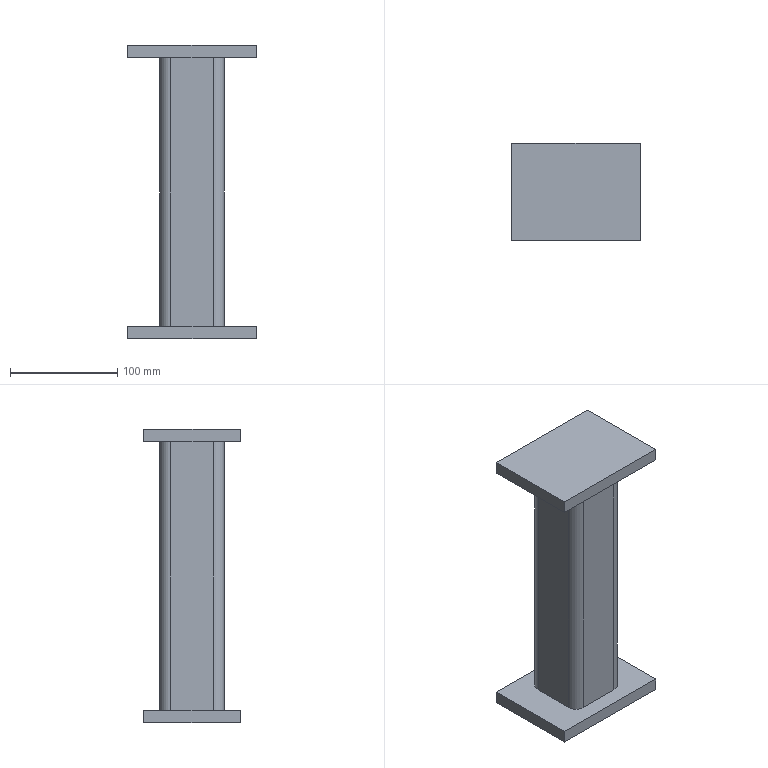Component | SolidWorks | 023-1 | 1 solid | 20 faces | box 120 x 90 x 274 mm | volume 1137740 mm3 | plane 16 | cylinder 4 | commonest cylinder face diameters 20 x4
build123d program:
from build123d import *

# Parameters (mm, degrees)
SKETCH1_W           = 120
SKETCH1_H           = 90
BOSS_EXTRUDE1_DEPTH = 12
SKETCH2_W           = 60
SKETCH2_H           = 60
BOSS_EXTRUDE2_DEPTH = 250
SKETCH4_W           = 120
SKETCH4_H           = 90
BOSS_EXTRUDE3_DEPTH = 12
FILLET1_R           = 10


with BuildPart() as part:
    # Sketch1 → Boss-Extrude1 (new body)
    with BuildSketch(Plane(origin=(0, 0, 0), x_dir=(1, 0, 0), z_dir=(0, 1, 0))):
        Rectangle(SKETCH1_W, SKETCH1_H)
    extrude(amount=BOSS_EXTRUDE1_DEPTH)

    # Sketch2 → Boss-Extrude2 (add)
    with BuildSketch(Plane(origin=(0, 12, 0), x_dir=(1, 0, 0), z_dir=(0, 1, 0))):
        Rectangle(SKETCH2_W, SKETCH2_H)
    extrude(amount=BOSS_EXTRUDE2_DEPTH)

    # Sketch4 → Boss-Extrude3 (add)
    with BuildSketch(Plane(origin=(0, 262, 0), x_dir=(1, 0, 0), z_dir=(0, 1, 0))):
        Rectangle(SKETCH4_W, SKETCH4_H)
    extrude(amount=BOSS_EXTRUDE3_DEPTH)

    # Fillet1
    fillet1_edges = [part.edges().sort_by_distance(p)[0] for p in [
        (30, 137, 30),
        (30, 137, -30),
        (-30, 137, -30),
        (-30, 137, 30),
    ]]
    fillet(fillet1_edges, radius=FILLET1_R)


solid = part.part

# Placed as in the assembly
solid = solid.moved(Location((-240.455, -60.942, -129.304), (90, 0, 0)))